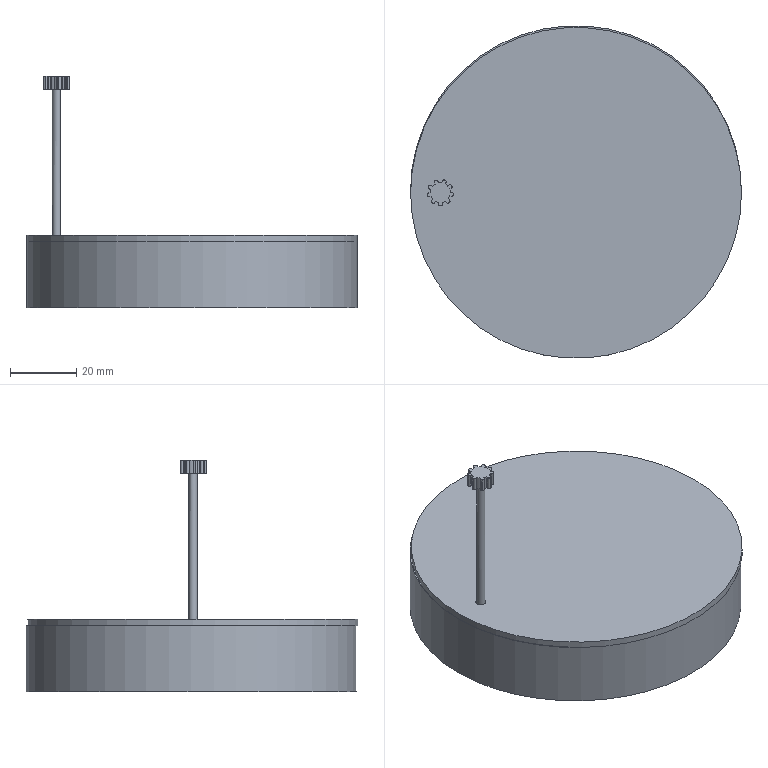Assembly | NX | mm | 14 component files | 15 solids | 661 faces | box 100.03 x 100.55 x 70 mm | volume 68786 mm3 | cylinder 421 | plane 240 | commonest cylinder face diameters 1 x179 21 x80 18 x80 5.5 x15 0.8 x12 5 x10 8 x9 6 x9
Bill of materials:
unnamed part 1 | 1 |  | Plain solid straight cylindrical rod with flat ends.
unnamed part 2 | 1 |  | Toothed wheel with about 20 rounded rectangular radial teeth and a raised cylindrical hub on one face. The hub has a small radial cross hole.
unnamed part 3 | 1 |  | Thin circular disk with a slight step on one face and one small through hole near the edge.
unnamed part 4 | 3 |  | Toothed wheel with about 20 rounded rectangular radial teeth and a large central through bore. It has no hub.
unnamed part 5 | 1 |  | Long, thin, flat link bar with fully rounded ends and one round through hole at each end.
unnamed part 6 | 1 |  | Shallow, open-top cylindrical tray with a thin wall and a flat floor. Several small cylindrical pins of different heights stand on the inside floor.
unnamed part 7 | 1 |  | Short, flat link plate with rounded ends and two large round through holes, one at each end.
unnamed part 8 | 2 |  | Solid flanged cylinder shaped like a plug or stepped pin: a thin, wider round head on a narrower cylindrical body.
unnamed part 9 | 1 |  | Thick, flat, obround plate with two large round through holes. Small cross holes drilled through the side wall break into one of the large holes.
unnamed part 10 | 1 |  | Long, thin, flat link bar with fully rounded ends and one round through hole at each end.
unnamed part 11 | 1 |  | Slender shaft with a small toothed (lobed) section at each end: a shorter, larger-diameter toothed head at one end and a longer, smaller toothed section at the other.
Mates:
1. fix | base 1 component
2. concentric | leadscrew 1 edge | base 1 edge
3. concentric | crank_rocker_4 1 edge | crank_rocker_1 1 edge
4. concentric | crank_rocker_2 1 edge | crank_rocker_4 1 edge
5. concentric | crank_rocker_2 1 edge | crank_rocker_3 1 edge
6. align lock | crank_rocker_3_fixed 1 face | crank_rocker_3 1 face
7. fix | crank_rocker_1 1 component
8. concentric | gear 3 edge | base 1 edge
9. concentric | gear 1 edge | base 1 edge
10. concentric | gear 2 edge | base 1 edge
11. align lock | crank_rocker_3_fixed 1 face | gear_1 1 face
12. concentric | gear_1 1 edge | base 1 edge
13. distance | crank_rocker_3_fixed 1 face | gear_1 1 face
14. bond | gear_1 1 component | crank_rocker_3 1 component
15. concentric | crank_fixed 2 edge | crank_rocker_2 1 edge
16. concentric | crank_fixed 1 edge | crank_rocker_2 1 edge
17. align lock | leadscrew 1 face | base_cover 1 face